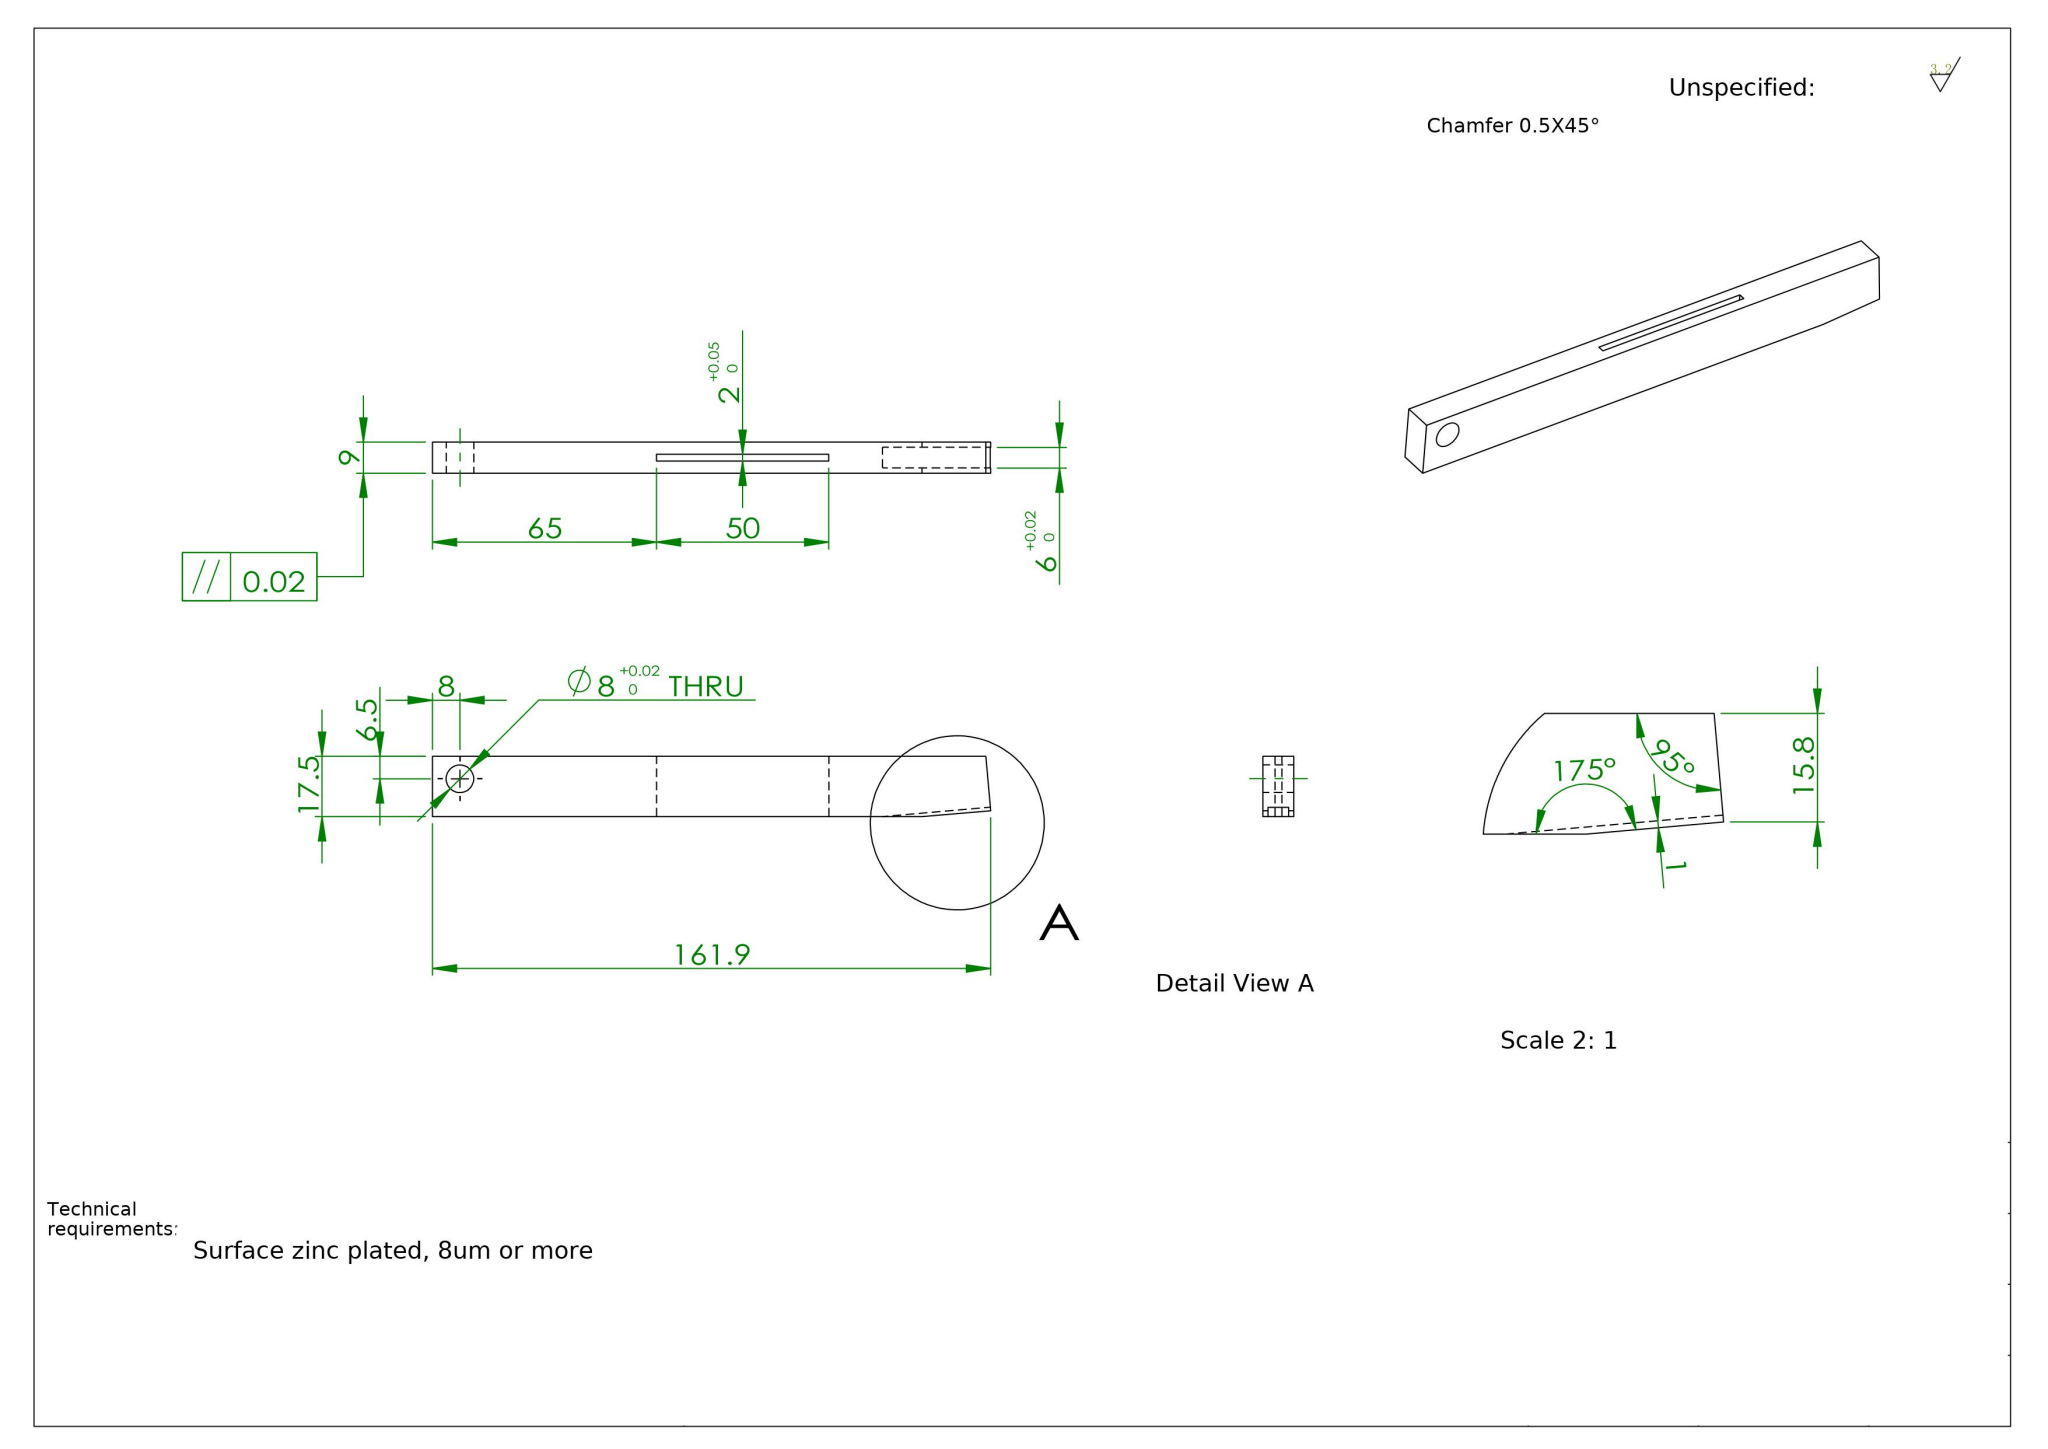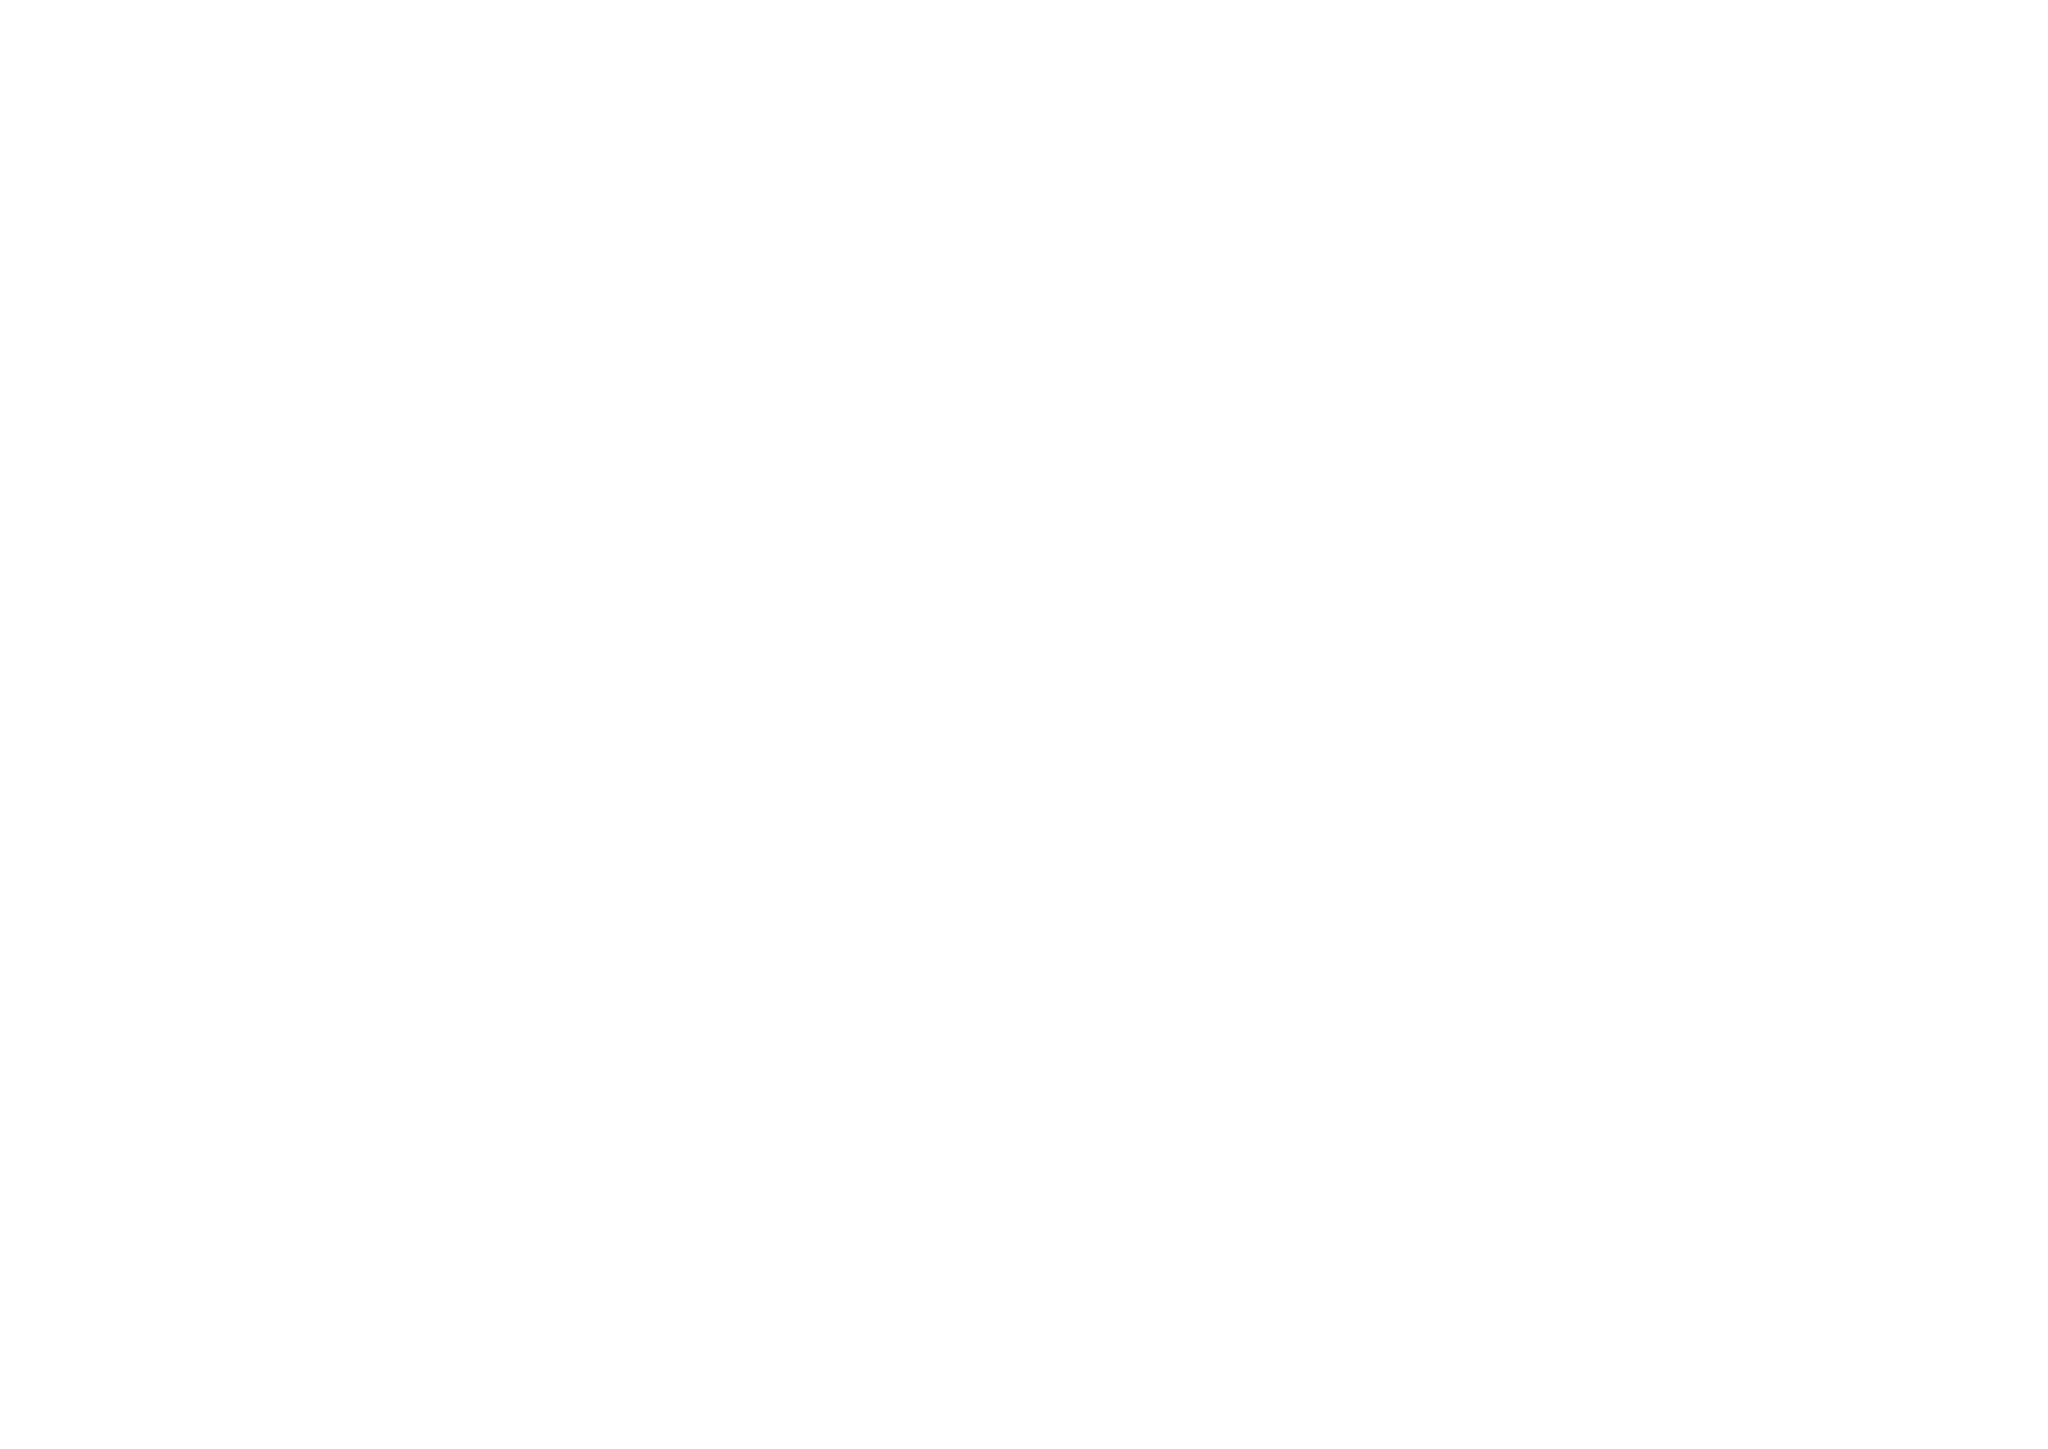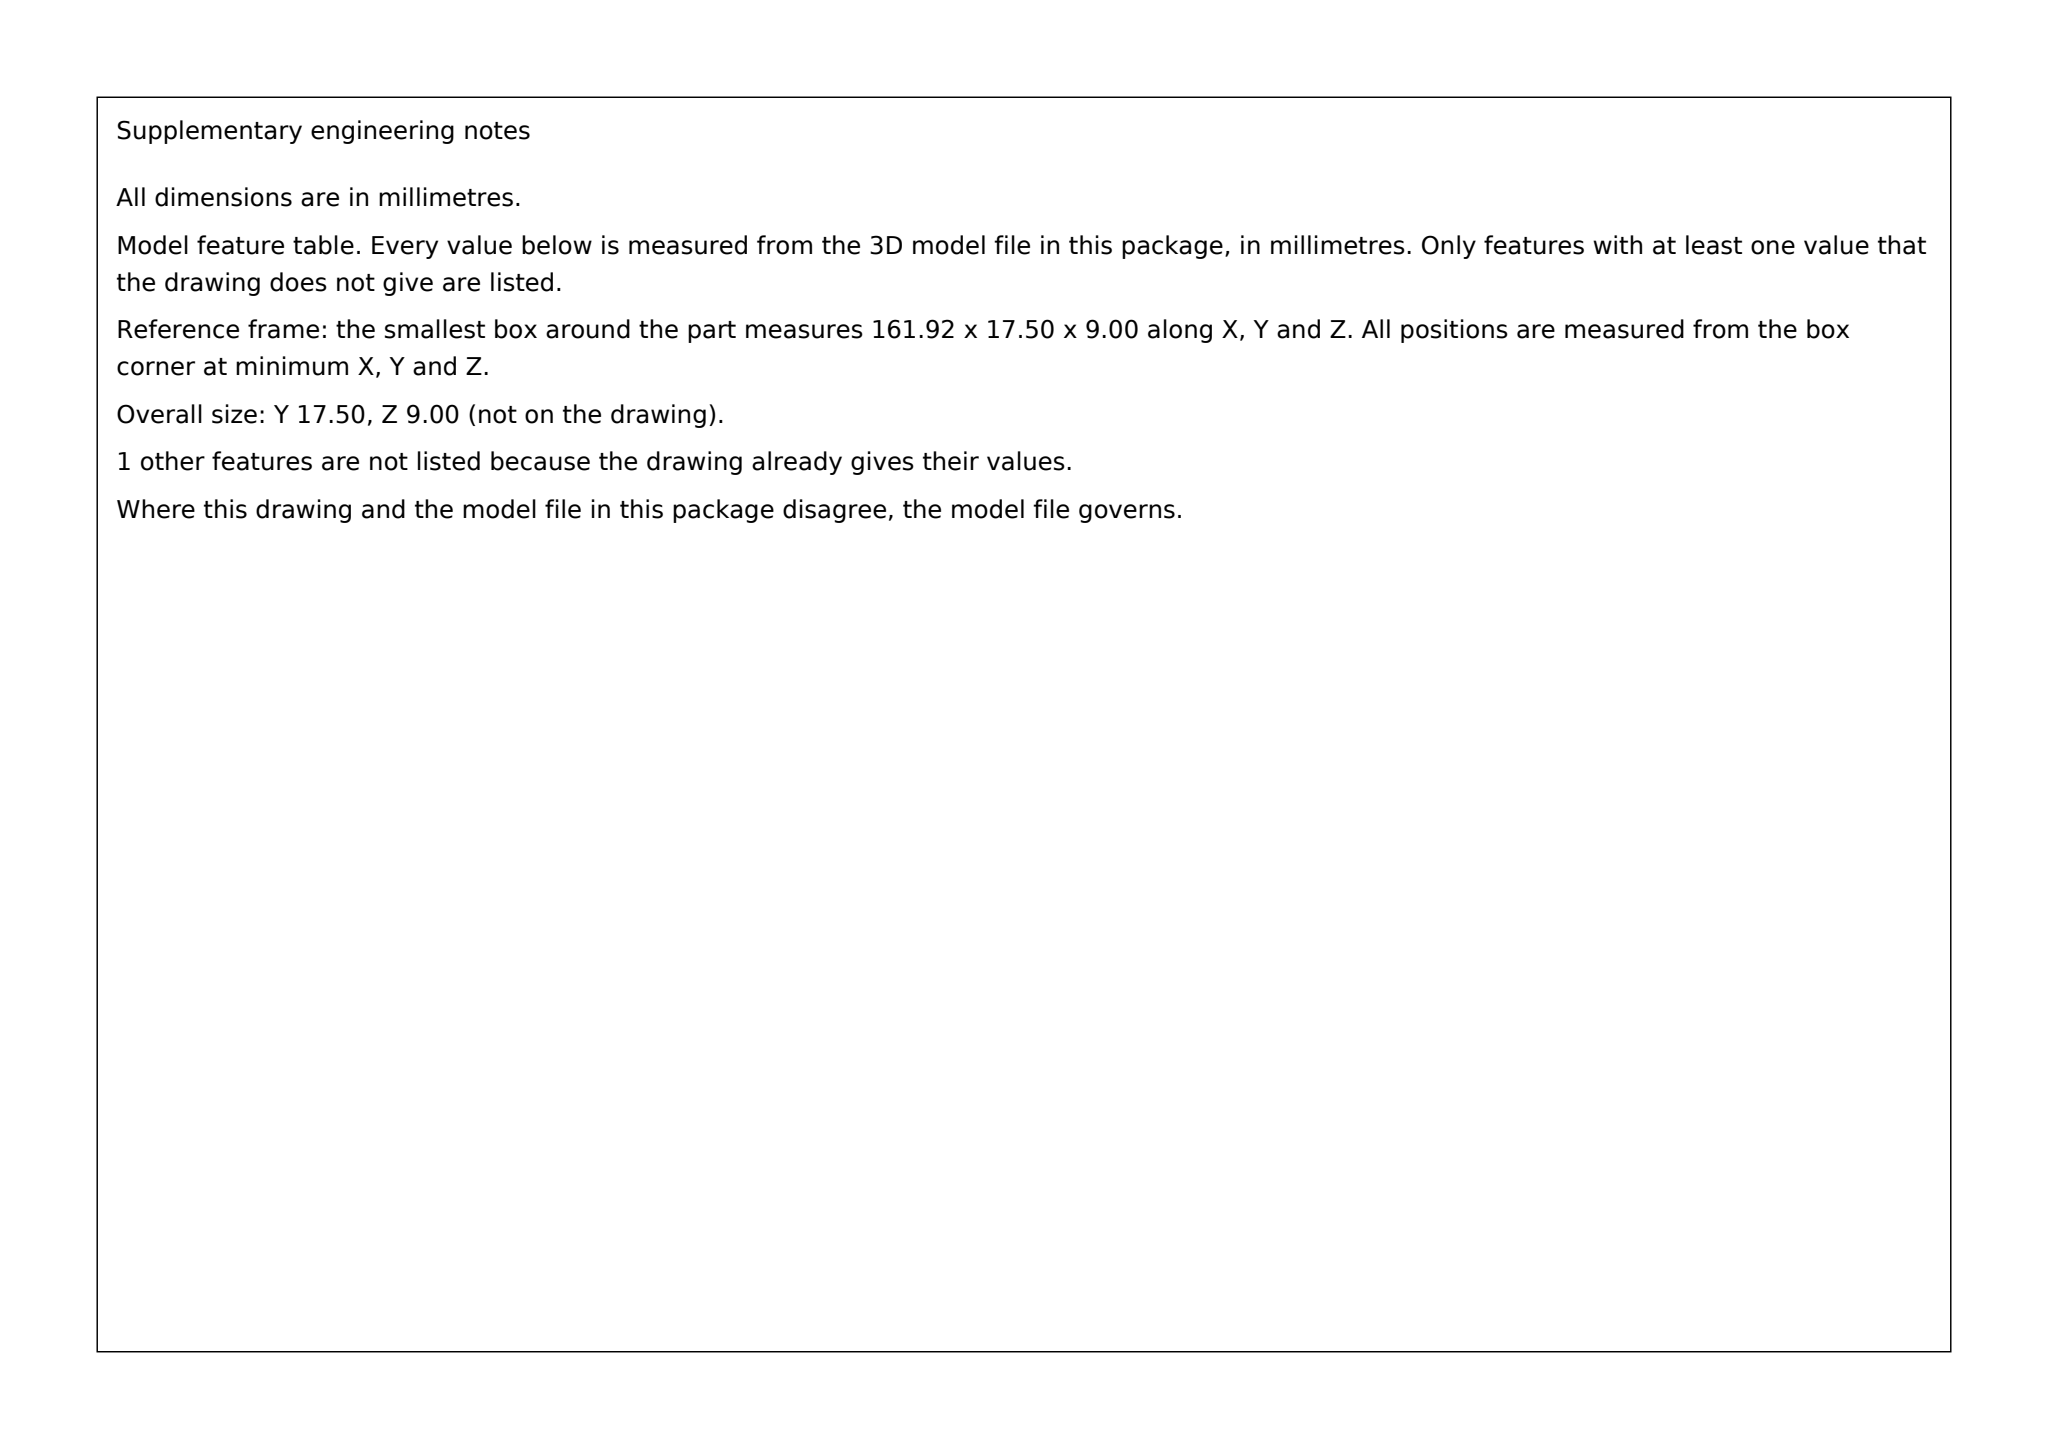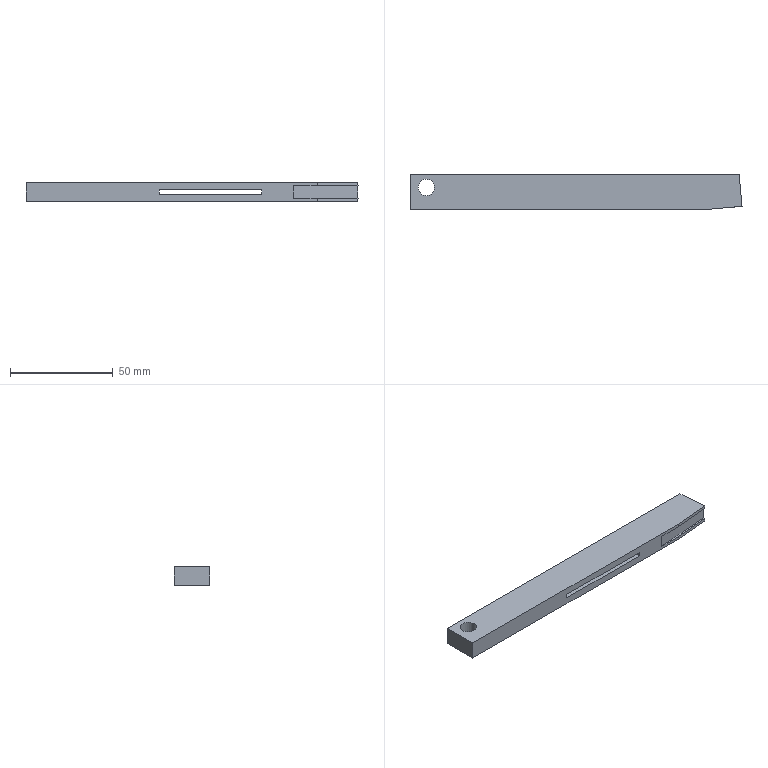Part | SolidWorks | mm | 1 solid | 17 faces | box 161.92 x 17.5 x 9 mm | volume 22892 mm3 | plane 15 | cylinder 2 | commonest cylinder face diameters 8 x2
STEP:
#1=CARTESIAN_POINT('',(4.,11.,-4.5));
#2=VERTEX_POINT('',#1);
#3=CARTESIAN_POINT('',(12.,11.,-4.5));
#4=VERTEX_POINT('',#3);
#5=CARTESIAN_POINT('',(8.,11.,-4.5));
#6=DIRECTION('',(0.,0.,1.));
#7=DIRECTION('',(1.,0.,0.));
#8=AXIS2_PLACEMENT_3D('',#5,#6,#7);
#9=CIRCLE('',#8,4.);
#10=EDGE_CURVE('',#2,#4,#9,.T.);
#11=ORIENTED_EDGE('',*,*,#10,.F.);
#12=CARTESIAN_POINT('',(4.,11.,4.5));
#13=VERTEX_POINT('',#12);
#14=CARTESIAN_POINT('',(4.,11.,-4.5));
#15=DIRECTION('',(0.,0.,1.));
#16=VECTOR('',#15,1000.);
#17=LINE('',#14,#16);
#18=EDGE_CURVE('',#2,#13,#17,.T.);
#19=ORIENTED_EDGE('',*,*,#18,.T.);
#20=CARTESIAN_POINT('',(12.,11.,4.5));
#21=VERTEX_POINT('',#20);
#22=CARTESIAN_POINT('',(8.,11.,4.5));
#23=DIRECTION('',(0.,0.,1.));
#24=DIRECTION('',(1.,0.,0.));
#25=AXIS2_PLACEMENT_3D('',#22,#23,#24);
#26=CIRCLE('',#25,4.);
#27=EDGE_CURVE('',#13,#21,#26,.T.);
#28=ORIENTED_EDGE('',*,*,#27,.T.);
#29=CARTESIAN_POINT('',(12.,11.,-4.5));
#30=DIRECTION('',(0.,0.,1.));
#31=VECTOR('',#30,1000.);
#32=LINE('',#29,#31);
#33=EDGE_CURVE('',#4,#21,#32,.T.);
#34=ORIENTED_EDGE('',*,*,#33,.F.);
#35=EDGE_LOOP('',(#11,#19,#28,#34));
#36=FACE_OUTER_BOUND('',#35,.T.);
#37=CARTESIAN_POINT('',(8.,11.,-4.5));
#38=DIRECTION('',(0.,0.,1.));
#39=DIRECTION('',(1.,0.,0.));
#40=AXIS2_PLACEMENT_3D('',#37,#38,#39);
#41=CYLINDRICAL_SURFACE('',#40,4.);
#42=ADVANCED_FACE('',(#36),#41,.F.);
#43=CARTESIAN_POINT('',(142.,0.,4.5));
#44=VERTEX_POINT('',#43);
#45=CARTESIAN_POINT('',(142.,-0.,3.));
#46=VERTEX_POINT('',#45);
#47=CARTESIAN_POINT('',(142.,0.,4.5));
#48=DIRECTION('',(0.,0.,-1.));
#49=VECTOR('',#48,1000.);
#50=LINE('',#47,#49);
#51=EDGE_CURVE('',#44,#46,#50,.T.);
#52=ORIENTED_EDGE('',*,*,#51,.T.);
#53=CARTESIAN_POINT('',(161.924,1.743,3.));
#54=VERTEX_POINT('',#53);
#55=CARTESIAN_POINT('',(120.338,-1.895,3.));
#56=DIRECTION('',(-0.9962,-0.08716,0.));
#57=VECTOR('',#56,1000.);
#58=LINE('',#55,#57);
#59=EDGE_CURVE('',#54,#46,#58,.T.);
#60=ORIENTED_EDGE('',*,*,#59,.F.);
#61=CARTESIAN_POINT('',(161.924,1.743,4.5));
#62=VERTEX_POINT('',#61);
#63=CARTESIAN_POINT('',(161.924,1.743,4.5));
#64=DIRECTION('',(0.,0.,-1.));
#65=VECTOR('',#64,1000.);
#66=LINE('',#63,#65);
#67=EDGE_CURVE('',#62,#54,#66,.T.);
#68=ORIENTED_EDGE('',*,*,#67,.F.);
#69=CARTESIAN_POINT('',(142.,0.,4.5));
#70=DIRECTION('',(0.9962,0.08716,0.));
#71=VECTOR('',#70,1000.);
#72=LINE('',#69,#71);
#73=EDGE_CURVE('',#44,#62,#72,.T.);
#74=ORIENTED_EDGE('',*,*,#73,.F.);
#75=EDGE_LOOP('',(#52,#60,#68,#74));
#76=FACE_OUTER_BOUND('',#75,.T.);
#77=CARTESIAN_POINT('',(142.,0.,4.5));
#78=DIRECTION('',(-0.08716,0.9962,0.));
#79=DIRECTION('',(-0.9962,-0.08716,0.));
#80=AXIS2_PLACEMENT_3D('',#77,#78,#79);
#81=PLANE('',#80);
#82=ADVANCED_FACE('',(#76),#81,.F.);
#83=CARTESIAN_POINT('',(115.,0.,-1.));
#84=VERTEX_POINT('',#83);
#85=CARTESIAN_POINT('',(65.,0.,-1.));
#86=VERTEX_POINT('',#85);
#87=CARTESIAN_POINT('',(65.,0.,-1.));
#88=DIRECTION('',(-1.,0.,0.));
#89=VECTOR('',#88,1000.);
#90=LINE('',#87,#89);
#91=EDGE_CURVE('',#84,#86,#90,.T.);
#92=ORIENTED_EDGE('',*,*,#91,.T.);
#93=CARTESIAN_POINT('',(65.,0.,1.));
#94=VERTEX_POINT('',#93);
#95=CARTESIAN_POINT('',(65.,0.,-1.));
#96=DIRECTION('',(0.,0.,1.));
#97=VECTOR('',#96,1000.);
#98=LINE('',#95,#97);
#99=EDGE_CURVE('',#86,#94,#98,.T.);
#100=ORIENTED_EDGE('',*,*,#99,.T.);
#101=CARTESIAN_POINT('',(115.,0.,1.));
#102=VERTEX_POINT('',#101);
#103=CARTESIAN_POINT('',(65.,0.,1.));
#104=DIRECTION('',(1.,0.,0.));
#105=VECTOR('',#104,1000.);
#106=LINE('',#103,#105);
#107=EDGE_CURVE('',#94,#102,#106,.T.);
#108=ORIENTED_EDGE('',*,*,#107,.T.);
#109=CARTESIAN_POINT('',(115.,0.,-1.));
#110=DIRECTION('',(0.,0.,-1.));
#111=VECTOR('',#110,1000.);
#112=LINE('',#109,#111);
#113=EDGE_CURVE('',#102,#84,#112,.T.);
#114=ORIENTED_EDGE('',*,*,#113,.T.);
#115=EDGE_LOOP('',(#92,#100,#108,#114));
#116=FACE_BOUND('',#115,.T.);
#117=CARTESIAN_POINT('',(130.526,0.,3.));
#118=VERTEX_POINT('',#117);
#119=CARTESIAN_POINT('',(130.526,0.,-3.));
#120=VERTEX_POINT('',#119);
#121=CARTESIAN_POINT('',(130.526,0.,4.5));
#122=DIRECTION('',(0.,0.,-1.));
#123=VECTOR('',#122,1000.);
#124=LINE('',#121,#123);
#125=EDGE_CURVE('',#118,#120,#124,.T.);
#126=ORIENTED_EDGE('',*,*,#125,.F.);
#127=CARTESIAN_POINT('',(0.,0.,3.));
#128=DIRECTION('',(1.,0.,0.));
#129=VECTOR('',#128,1000.);
#130=LINE('',#127,#129);
#131=EDGE_CURVE('',#118,#46,#130,.T.);
#132=ORIENTED_EDGE('',*,*,#131,.T.);
#133=ORIENTED_EDGE('',*,*,#51,.F.);
#134=CARTESIAN_POINT('',(0.,0.,4.5));
#135=VERTEX_POINT('',#134);
#136=CARTESIAN_POINT('',(0.,0.,4.5));
#137=DIRECTION('',(1.,0.,0.));
#138=VECTOR('',#137,1000.);
#139=LINE('',#136,#138);
#140=EDGE_CURVE('',#135,#44,#139,.T.);
#141=ORIENTED_EDGE('',*,*,#140,.F.);
#142=CARTESIAN_POINT('',(0.,0.,-4.5));
#143=VERTEX_POINT('',#142);
#144=CARTESIAN_POINT('',(0.,0.,4.5));
#145=DIRECTION('',(0.,0.,-1.));
#146=VECTOR('',#145,1000.);
#147=LINE('',#144,#146);
#148=EDGE_CURVE('',#135,#143,#147,.T.);
#149=ORIENTED_EDGE('',*,*,#148,.T.);
#150=CARTESIAN_POINT('',(142.,0.,-4.5));
#151=VERTEX_POINT('',#150);
#152=CARTESIAN_POINT('',(0.,0.,-4.5));
#153=DIRECTION('',(1.,0.,0.));
#154=VECTOR('',#153,1000.);
#155=LINE('',#152,#154);
#156=EDGE_CURVE('',#143,#151,#155,.T.);
#157=ORIENTED_EDGE('',*,*,#156,.T.);
#158=CARTESIAN_POINT('',(142.,-0.,-3.));
#159=VERTEX_POINT('',#158);
#160=CARTESIAN_POINT('',(142.,0.,4.5));
#161=DIRECTION('',(0.,0.,-1.));
#162=VECTOR('',#161,1000.);
#163=LINE('',#160,#162);
#164=EDGE_CURVE('',#159,#151,#163,.T.);
#165=ORIENTED_EDGE('',*,*,#164,.F.);
#166=CARTESIAN_POINT('',(0.,0.,-3.));
#167=DIRECTION('',(-1.,0.,0.));
#168=VECTOR('',#167,1000.);
#169=LINE('',#166,#168);
#170=EDGE_CURVE('',#159,#120,#169,.T.);
#171=ORIENTED_EDGE('',*,*,#170,.T.);
#172=EDGE_LOOP('',(#126,#132,#133,#141,#149,#157,#165,#171));
#173=FACE_OUTER_BOUND('',#172,.T.);
#174=CARTESIAN_POINT('',(0.,0.,4.5));
#175=DIRECTION('',(0.,1.,0.));
#176=DIRECTION('',(0.,0.,1.));
#177=AXIS2_PLACEMENT_3D('',#174,#175,#176);
#178=PLANE('',#177);
#179=ADVANCED_FACE('',(#116,#173),#178,.F.);
#180=CARTESIAN_POINT('',(161.924,1.743,-3.));
#181=VERTEX_POINT('',#180);
#182=CARTESIAN_POINT('',(161.924,1.743,-4.5));
#183=VERTEX_POINT('',#182);
#184=CARTESIAN_POINT('',(161.924,1.743,4.5));
#185=DIRECTION('',(0.,0.,-1.));
#186=VECTOR('',#185,1000.);
#187=LINE('',#184,#186);
#188=EDGE_CURVE('',#181,#183,#187,.T.);
#189=ORIENTED_EDGE('',*,*,#188,.F.);
#190=CARTESIAN_POINT('',(120.338,-1.895,-3.));
#191=DIRECTION('',(0.9962,0.08716,0.));
#192=VECTOR('',#191,1000.);
#193=LINE('',#190,#192);
#194=EDGE_CURVE('',#159,#181,#193,.T.);
#195=ORIENTED_EDGE('',*,*,#194,.F.);
#196=ORIENTED_EDGE('',*,*,#164,.T.);
#197=CARTESIAN_POINT('',(142.,0.,-4.5));
#198=DIRECTION('',(0.9962,0.08716,0.));
#199=VECTOR('',#198,1000.);
#200=LINE('',#197,#199);
#201=EDGE_CURVE('',#151,#183,#200,.T.);
#202=ORIENTED_EDGE('',*,*,#201,.T.);
#203=EDGE_LOOP('',(#189,#195,#196,#202));
#204=FACE_OUTER_BOUND('',#203,.T.);
#205=CARTESIAN_POINT('',(142.,0.,4.5));
#206=DIRECTION('',(-0.08716,0.9962,0.));
#207=DIRECTION('',(-0.9962,-0.08716,0.));
#208=AXIS2_PLACEMENT_3D('',#205,#206,#207);
#209=PLANE('',#208);
#210=ADVANCED_FACE('',(#204),#209,.F.);
#211=ORIENTED_EDGE('',*,*,#67,.T.);
#212=CARTESIAN_POINT('',(161.837,2.739,3.));
#213=VERTEX_POINT('',#212);
#214=CARTESIAN_POINT('',(161.837,2.739,3.));
#215=DIRECTION('',(0.08716,-0.9962,0.));
#216=VECTOR('',#215,1000.);
#217=LINE('',#214,#216);
#218=EDGE_CURVE('',#213,#54,#217,.T.);
#219=ORIENTED_EDGE('',*,*,#218,.F.);
#220=CARTESIAN_POINT('',(161.837,2.739,-3.));
#221=VERTEX_POINT('',#220);
#222=CARTESIAN_POINT('',(161.837,2.739,3.));
#223=DIRECTION('',(0.,0.,1.));
#224=VECTOR('',#223,1000.);
#225=LINE('',#222,#224);
#226=EDGE_CURVE('',#221,#213,#225,.T.);
#227=ORIENTED_EDGE('',*,*,#226,.F.);
#228=CARTESIAN_POINT('',(161.837,2.739,-3.));
#229=DIRECTION('',(0.08716,-0.9962,0.));
#230=VECTOR('',#229,1000.);
#231=LINE('',#228,#230);
#232=EDGE_CURVE('',#221,#181,#231,.T.);
#233=ORIENTED_EDGE('',*,*,#232,.T.);
#234=ORIENTED_EDGE('',*,*,#188,.T.);
#235=CARTESIAN_POINT('',(160.545,17.5,-4.5));
#236=VERTEX_POINT('',#235);
#237=CARTESIAN_POINT('',(160.545,17.5,-4.5));
#238=DIRECTION('',(-0.08716,0.9962,0.));
#239=VECTOR('',#238,1000.);
#240=LINE('',#237,#239);
#241=EDGE_CURVE('',#183,#236,#240,.T.);
#242=ORIENTED_EDGE('',*,*,#241,.T.);
#243=CARTESIAN_POINT('',(160.545,17.5,4.5));
#244=VERTEX_POINT('',#243);
#245=CARTESIAN_POINT('',(160.545,17.5,4.5));
#246=DIRECTION('',(0.,0.,-1.));
#247=VECTOR('',#246,1000.);
#248=LINE('',#245,#247);
#249=EDGE_CURVE('',#244,#236,#248,.T.);
#250=ORIENTED_EDGE('',*,*,#249,.F.);
#251=CARTESIAN_POINT('',(160.545,17.5,4.5));
#252=DIRECTION('',(-0.08716,0.9962,0.));
#253=VECTOR('',#252,1000.);
#254=LINE('',#251,#253);
#255=EDGE_CURVE('',#62,#244,#254,.T.);
#256=ORIENTED_EDGE('',*,*,#255,.F.);
#257=EDGE_LOOP('',(#211,#219,#227,#233,#234,#242,#250,#256));
#258=FACE_OUTER_BOUND('',#257,.T.);
#259=CARTESIAN_POINT('',(160.545,17.5,4.5));
#260=DIRECTION('',(-0.9962,-0.08716,0.));
#261=DIRECTION('',(0.08716,-0.9962,0.));
#262=AXIS2_PLACEMENT_3D('',#259,#260,#261);
#263=PLANE('',#262);
#264=ADVANCED_FACE('',(#258),#263,.F.);
#265=CARTESIAN_POINT('',(65.,17.5,1.));
#266=VERTEX_POINT('',#265);
#267=CARTESIAN_POINT('',(115.,17.5,1.));
#268=VERTEX_POINT('',#267);
#269=CARTESIAN_POINT('',(65.,17.5,1.));
#270=DIRECTION('',(1.,0.,0.));
#271=VECTOR('',#270,1000.);
#272=LINE('',#269,#271);
#273=EDGE_CURVE('',#266,#268,#272,.T.);
#274=ORIENTED_EDGE('',*,*,#273,.F.);
#275=CARTESIAN_POINT('',(65.,17.5,-1.));
#276=VERTEX_POINT('',#275);
#277=CARTESIAN_POINT('',(65.,17.5,-1.));
#278=DIRECTION('',(0.,0.,1.));
#279=VECTOR('',#278,1000.);
#280=LINE('',#277,#279);
#281=EDGE_CURVE('',#276,#266,#280,.T.);
#282=ORIENTED_EDGE('',*,*,#281,.F.);
#283=CARTESIAN_POINT('',(115.,17.5,-1.));
#284=VERTEX_POINT('',#283);
#285=CARTESIAN_POINT('',(65.,17.5,-1.));
#286=DIRECTION('',(-1.,0.,0.));
#287=VECTOR('',#286,1000.);
#288=LINE('',#285,#287);
#289=EDGE_CURVE('',#284,#276,#288,.T.);
#290=ORIENTED_EDGE('',*,*,#289,.F.);
#291=CARTESIAN_POINT('',(115.,17.5,-1.));
#292=DIRECTION('',(0.,0.,-1.));
#293=VECTOR('',#292,1000.);
#294=LINE('',#291,#293);
#295=EDGE_CURVE('',#268,#284,#294,.T.);
#296=ORIENTED_EDGE('',*,*,#295,.F.);
#297=EDGE_LOOP('',(#274,#282,#290,#296));
#298=FACE_BOUND('',#297,.T.);
#299=CARTESIAN_POINT('',(0.,17.5,-4.5));
#300=VERTEX_POINT('',#299);
#301=CARTESIAN_POINT('',(0.,17.5,-4.5));
#302=DIRECTION('',(-1.,0.,0.));
#303=VECTOR('',#302,1000.);
#304=LINE('',#301,#303);
#305=EDGE_CURVE('',#236,#300,#304,.T.);
#306=ORIENTED_EDGE('',*,*,#305,.T.);
#307=CARTESIAN_POINT('',(0.,17.5,4.5));
#308=VERTEX_POINT('',#307);
#309=CARTESIAN_POINT('',(0.,17.5,4.5));
#310=DIRECTION('',(0.,0.,-1.));
#311=VECTOR('',#310,1000.);
#312=LINE('',#309,#311);
#313=EDGE_CURVE('',#308,#300,#312,.T.);
#314=ORIENTED_EDGE('',*,*,#313,.F.);
#315=CARTESIAN_POINT('',(0.,17.5,4.5));
#316=DIRECTION('',(-1.,0.,0.));
#317=VECTOR('',#316,1000.);
#318=LINE('',#315,#317);
#319=EDGE_CURVE('',#244,#308,#318,.T.);
#320=ORIENTED_EDGE('',*,*,#319,.F.);
#321=ORIENTED_EDGE('',*,*,#249,.T.);
#322=EDGE_LOOP('',(#306,#314,#320,#321));
#323=FACE_OUTER_BOUND('',#322,.T.);
#324=CARTESIAN_POINT('',(0.,17.5,4.5));
#325=DIRECTION('',(0.,-1.,0.));
#326=DIRECTION('',(0.,0.,-1.));
#327=AXIS2_PLACEMENT_3D('',#324,#325,#326);
#328=PLANE('',#327);
#329=ADVANCED_FACE('',(#298,#323),#328,.F.);
#330=CARTESIAN_POINT('',(0.,0.,-4.5));
#331=DIRECTION('',(-0.,-1.,0.));
#332=VECTOR('',#331,1000.);
#333=LINE('',#330,#332);
#334=EDGE_CURVE('',#300,#143,#333,.T.);
#335=ORIENTED_EDGE('',*,*,#334,.T.);
#336=ORIENTED_EDGE('',*,*,#148,.F.);
#337=CARTESIAN_POINT('',(0.,0.,4.5));
#338=DIRECTION('',(-0.,-1.,0.));
#339=VECTOR('',#338,1000.);
#340=LINE('',#337,#339);
#341=EDGE_CURVE('',#308,#135,#340,.T.);
#342=ORIENTED_EDGE('',*,*,#341,.F.);
#343=ORIENTED_EDGE('',*,*,#313,.T.);
#344=EDGE_LOOP('',(#335,#336,#342,#343));
#345=FACE_OUTER_BOUND('',#344,.T.);
#346=CARTESIAN_POINT('',(0.,0.,4.5));
#347=DIRECTION('',(1.,-0.,0.));
#348=DIRECTION('',(0.,1.,0.));
#349=AXIS2_PLACEMENT_3D('',#346,#347,#348);
#350=PLANE('',#349);
#351=ADVANCED_FACE('',(#345),#350,.F.);
#352=CARTESIAN_POINT('',(8.,11.,4.5));
#353=DIRECTION('',(0.,0.,1.));
#354=DIRECTION('',(1.,0.,0.));
#355=AXIS2_PLACEMENT_3D('',#352,#353,#354);
#356=CIRCLE('',#355,4.);
#357=EDGE_CURVE('',#21,#13,#356,.T.);
#358=ORIENTED_EDGE('',*,*,#357,.F.);
#359=ORIENTED_EDGE('',*,*,#27,.F.);
#360=EDGE_LOOP('',(#358,#359));
#361=FACE_BOUND('',#360,.T.);
#362=ORIENTED_EDGE('',*,*,#140,.T.);
#363=ORIENTED_EDGE('',*,*,#73,.T.);
#364=ORIENTED_EDGE('',*,*,#255,.T.);
#365=ORIENTED_EDGE('',*,*,#319,.T.);
#366=ORIENTED_EDGE('',*,*,#341,.T.);
#367=EDGE_LOOP('',(#362,#363,#364,#365,#366));
#368=FACE_OUTER_BOUND('',#367,.T.);
#369=CARTESIAN_POINT('',(0.,0.,4.5));
#370=DIRECTION('',(0.,0.,1.));
#371=DIRECTION('',(1.,0.,0.));
#372=AXIS2_PLACEMENT_3D('',#369,#370,#371);
#373=PLANE('',#372);
#374=ADVANCED_FACE('',(#361,#368),#373,.T.);
#375=CARTESIAN_POINT('',(8.,11.,-4.5));
#376=DIRECTION('',(0.,0.,1.));
#377=DIRECTION('',(1.,0.,0.));
#378=AXIS2_PLACEMENT_3D('',#375,#376,#377);
#379=CIRCLE('',#378,4.);
#380=EDGE_CURVE('',#4,#2,#379,.T.);
#381=ORIENTED_EDGE('',*,*,#380,.T.);
#382=ORIENTED_EDGE('',*,*,#10,.T.);
#383=EDGE_LOOP('',(#381,#382));
#384=FACE_BOUND('',#383,.T.);
#385=ORIENTED_EDGE('',*,*,#156,.F.);
#386=ORIENTED_EDGE('',*,*,#334,.F.);
#387=ORIENTED_EDGE('',*,*,#305,.F.);
#388=ORIENTED_EDGE('',*,*,#241,.F.);
#389=ORIENTED_EDGE('',*,*,#201,.F.);
#390=EDGE_LOOP('',(#385,#386,#387,#388,#389));
#391=FACE_OUTER_BOUND('',#390,.T.);
#392=CARTESIAN_POINT('',(0.,0.,-4.5));
#393=DIRECTION('',(0.,0.,1.));
#394=DIRECTION('',(1.,0.,0.));
#395=AXIS2_PLACEMENT_3D('',#392,#393,#394);
#396=PLANE('',#395);
#397=ADVANCED_FACE('',(#384,#391),#396,.F.);
#398=ORIENTED_EDGE('',*,*,#18,.F.);
#399=ORIENTED_EDGE('',*,*,#380,.F.);
#400=ORIENTED_EDGE('',*,*,#33,.T.);
#401=ORIENTED_EDGE('',*,*,#357,.T.);
#402=EDGE_LOOP('',(#398,#399,#400,#401));
#403=FACE_OUTER_BOUND('',#402,.T.);
#404=CARTESIAN_POINT('',(8.,11.,-4.5));
#405=DIRECTION('',(0.,0.,1.));
#406=DIRECTION('',(1.,0.,0.));
#407=AXIS2_PLACEMENT_3D('',#404,#405,#406);
#408=CYLINDRICAL_SURFACE('',#407,4.);
#409=ADVANCED_FACE('',(#403),#408,.F.);
#410=ORIENTED_EDGE('',*,*,#281,.T.);
#411=CARTESIAN_POINT('',(65.,0.,1.));
#412=DIRECTION('',(0.,1.,0.));
#413=VECTOR('',#412,1000.);
#414=LINE('',#411,#413);
#415=EDGE_CURVE('',#94,#266,#414,.T.);
#416=ORIENTED_EDGE('',*,*,#415,.F.);
#417=ORIENTED_EDGE('',*,*,#99,.F.);
#418=CARTESIAN_POINT('',(65.,0.,-1.));
#419=DIRECTION('',(0.,1.,0.));
#420=VECTOR('',#419,1000.);
#421=LINE('',#418,#420);
#422=EDGE_CURVE('',#86,#276,#421,.T.);
#423=ORIENTED_EDGE('',*,*,#422,.T.);
#424=EDGE_LOOP('',(#410,#416,#417,#423));
#425=FACE_OUTER_BOUND('',#424,.T.);
#426=CARTESIAN_POINT('',(65.,0.,-1.));
#427=DIRECTION('',(-1.,0.,0.));
#428=DIRECTION('',(0.,0.,1.));
#429=AXIS2_PLACEMENT_3D('',#426,#427,#428);
#430=PLANE('',#429);
#431=ADVANCED_FACE('',(#425),#430,.F.);
#432=ORIENTED_EDGE('',*,*,#289,.T.);
#433=ORIENTED_EDGE('',*,*,#422,.F.);
#434=ORIENTED_EDGE('',*,*,#91,.F.);
#435=CARTESIAN_POINT('',(115.,0.,-1.));
#436=DIRECTION('',(0.,1.,0.));
#437=VECTOR('',#436,1000.);
#438=LINE('',#435,#437);
#439=EDGE_CURVE('',#84,#284,#438,.T.);
#440=ORIENTED_EDGE('',*,*,#439,.T.);
#441=EDGE_LOOP('',(#432,#433,#434,#440));
#442=FACE_OUTER_BOUND('',#441,.T.);
#443=CARTESIAN_POINT('',(65.,0.,-1.));
#444=DIRECTION('',(0.,0.,-1.));
#445=DIRECTION('',(-1.,0.,0.));
#446=AXIS2_PLACEMENT_3D('',#443,#444,#445);
#447=PLANE('',#446);
#448=ADVANCED_FACE('',(#442),#447,.F.);
#449=ORIENTED_EDGE('',*,*,#295,.T.);
#450=ORIENTED_EDGE('',*,*,#439,.F.);
#451=ORIENTED_EDGE('',*,*,#113,.F.);
#452=CARTESIAN_POINT('',(115.,0.,1.));
#453=DIRECTION('',(0.,1.,0.));
#454=VECTOR('',#453,1000.);
#455=LINE('',#452,#454);
#456=EDGE_CURVE('',#102,#268,#455,.T.);
#457=ORIENTED_EDGE('',*,*,#456,.T.);
#458=EDGE_LOOP('',(#449,#450,#451,#457));
#459=FACE_OUTER_BOUND('',#458,.T.);
#460=CARTESIAN_POINT('',(115.,0.,-1.));
#461=DIRECTION('',(1.,0.,0.));
#462=DIRECTION('',(0.,0.,-1.));
#463=AXIS2_PLACEMENT_3D('',#460,#461,#462);
#464=PLANE('',#463);
#465=ADVANCED_FACE('',(#459),#464,.F.);
#466=ORIENTED_EDGE('',*,*,#273,.T.);
#467=ORIENTED_EDGE('',*,*,#456,.F.);
#468=ORIENTED_EDGE('',*,*,#107,.F.);
#469=ORIENTED_EDGE('',*,*,#415,.T.);
#470=EDGE_LOOP('',(#466,#467,#468,#469));
#471=FACE_OUTER_BOUND('',#470,.T.);
#472=CARTESIAN_POINT('',(65.,0.,1.));
#473=DIRECTION('',(0.,0.,1.));
#474=DIRECTION('',(1.,0.,0.));
#475=AXIS2_PLACEMENT_3D('',#472,#473,#474);
#476=PLANE('',#475);
#477=ADVANCED_FACE('',(#471),#476,.F.);
#478=CARTESIAN_POINT('',(120.251,-0.8989,3.));
#479=DIRECTION('',(-0.9962,-0.08716,0.));
#480=VECTOR('',#479,1000.);
#481=LINE('',#478,#480);
#482=EDGE_CURVE('',#213,#118,#481,.T.);
#483=ORIENTED_EDGE('',*,*,#482,.F.);
#484=ORIENTED_EDGE('',*,*,#218,.T.);
#485=ORIENTED_EDGE('',*,*,#59,.T.);
#486=ORIENTED_EDGE('',*,*,#131,.F.);
#487=EDGE_LOOP('',(#483,#484,#485,#486));
#488=FACE_OUTER_BOUND('',#487,.T.);
#489=CARTESIAN_POINT('',(120.251,-0.8989,3.));
#490=DIRECTION('',(0.,0.,1.));
#491=DIRECTION('',(1.,0.,0.));
#492=AXIS2_PLACEMENT_3D('',#489,#490,#491);
#493=PLANE('',#492);
#494=ADVANCED_FACE('',(#488),#493,.F.);
#495=ORIENTED_EDGE('',*,*,#194,.T.);
#496=ORIENTED_EDGE('',*,*,#232,.F.);
#497=CARTESIAN_POINT('',(120.251,-0.8989,-3.));
#498=DIRECTION('',(0.9962,0.08716,0.));
#499=VECTOR('',#498,1000.);
#500=LINE('',#497,#499);
#501=EDGE_CURVE('',#120,#221,#500,.T.);
#502=ORIENTED_EDGE('',*,*,#501,.F.);
#503=ORIENTED_EDGE('',*,*,#170,.F.);
#504=EDGE_LOOP('',(#495,#496,#502,#503));
#505=FACE_OUTER_BOUND('',#504,.T.);
#506=CARTESIAN_POINT('',(120.251,-0.8989,-3.));
#507=DIRECTION('',(0.,0.,-1.));
#508=DIRECTION('',(-1.,0.,0.));
#509=AXIS2_PLACEMENT_3D('',#506,#507,#508);
#510=PLANE('',#509);
#511=ADVANCED_FACE('',(#505),#510,.F.);
#512=ORIENTED_EDGE('',*,*,#125,.T.);
#513=ORIENTED_EDGE('',*,*,#501,.T.);
#514=ORIENTED_EDGE('',*,*,#226,.T.);
#515=ORIENTED_EDGE('',*,*,#482,.T.);
#516=EDGE_LOOP('',(#512,#513,#514,#515));
#517=FACE_OUTER_BOUND('',#516,.T.);
#518=CARTESIAN_POINT('',(120.251,-0.8989,-3.));
#519=DIRECTION('',(0.08716,-0.9962,0.));
#520=DIRECTION('',(0.9962,0.08716,0.));
#521=AXIS2_PLACEMENT_3D('',#518,#519,#520);
#522=PLANE('',#521);
#523=ADVANCED_FACE('',(#517),#522,.T.);
#524=CLOSED_SHELL('',(#42,#82,#179,#210,#264,#329,#351,#374,#397,#409,#431,#448,#465,#477,#494,#511,#523));
#525=MANIFOLD_SOLID_BREP('',#524);
#526=CARTESIAN_POINT('',(0.,0.,0.));
#527=DIRECTION('',(0.,0.,1.));
#528=DIRECTION('',(1.,0.,0.));
#529=AXIS2_PLACEMENT_3D('',#526,#527,#528);
#530=(LENGTH_UNIT()NAMED_UNIT(*)SI_UNIT(.MILLI.,.METRE.));
#531=UNCERTAINTY_MEASURE_WITH_UNIT(LENGTH_MEASURE(0.00001),#530,'','');
#532=(NAMED_UNIT(*)PLANE_ANGLE_UNIT()SI_UNIT($,.RADIAN.));
#533=(NAMED_UNIT(*)SI_UNIT($,.STERADIAN.)SOLID_ANGLE_UNIT());
#534=(GEOMETRIC_REPRESENTATION_CONTEXT(3)GLOBAL_UNCERTAINTY_ASSIGNED_CONTEXT((#531))GLOBAL_UNIT_ASSIGNED_CONTEXT((#530,#532,#533))REPRESENTATION_CONTEXT('',''));
#535=ADVANCED_BREP_SHAPE_REPRESENTATION('',(#525,#529),#534);